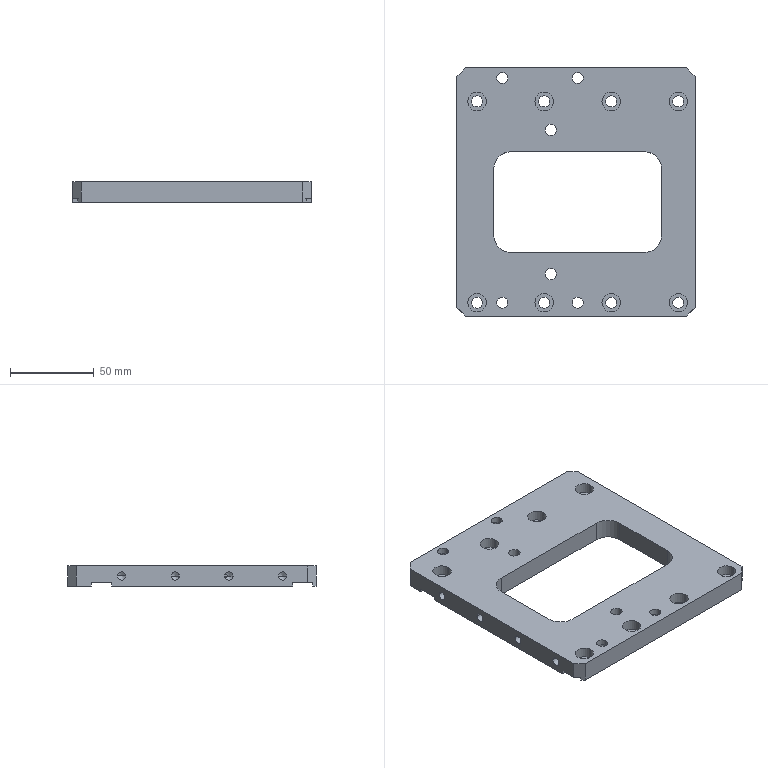Component | SolidWorks | 17081801-804-013A-1 | 1 solid | 106 faces | box 142 x 148 x 12 mm | volume 162736 mm3 | cylinder 64 | plane 34 | cone 8 | commonest cylinder face diameters 11 x24 6.6 x24 5 x8 6.8 x4 20 x4 | material AL6061
build123d program:
from build123d import *

# Parameters (mm, degrees)
SKETCH1_W                                       = 136
SKETCH1_H                                       = 140
BOSS_EXTRUDE1_DEPTH                             = 6
M6_HEX_SOCKET_HEAD_CAP_SCREW_CBORE1_D           = 6.6
M6_HEX_SOCKET_HEAD_CAP_SCREW_CBORE1_DEPTH       = 13
M6_HEX_SOCKET_HEAD_CAP_SCREW_CBORE1_CBORE_D     = 11
M6_HEX_SOCKET_HEAD_CAP_SCREW_CBORE1_CBORE_DEPTH = 6.4
M6_HEX_SOCKET_HEAD_CAP_SCREW_CBORE1_TIP         = 1.983
SKETCH12_W                                      = 136
SKETCH12_H                                      = 12
BOSS_EXTRUDE2_DEPTH                             = 2
M6_TAPPED_HOLE1_D                               = 5
M6_TAPPED_HOLE1_DEPTH                           = 13
M6_TAPPED_HOLE1_TIP                             = 1.502
SKETCH9_W                                       = 12
SKETCH9_H                                       = 180
CUT_EXTRUDE2_DEPTH                              = 2
SKETCH13_W                                      = 142
SKETCH13_H                                      = 12
BOSS_EXTRUDE3_DEPTH                             = 12
M6_HEX_SOCKET_HEAD_CAP_SCREW_CBORE2_AT_2_COUNT  = 2
M6_HEX_SOCKET_HEAD_CAP_SCREW_CBORE2_AT_2_PITCH  = 134
LPATTERN1_COUNT                                 = 2
LPATTERN1_PITCH                                 = 45
SKETCH8_W                                       = 60
SKETCH8_H                                       = 100
CUT_EXTRUDE1_DEPTH                              = 109.296
FILLET1_R                                       = 10
CHAMFER3_SIZE                                   = 5
M8_TAPPED_HOLE1_D                               = 6.8


with BuildPart() as part:
    # Sketch1 → Boss-Extrude1 (new, symmetric)
    with BuildSketch(Plane(origin=(0, 0, 0), x_dir=(1, 0, 0), z_dir=(0, 1, 0))):
        Rectangle(SKETCH1_W, SKETCH1_H)
    extrude(amount=BOSS_EXTRUDE1_DEPTH, both=True)

    # M6 Hex Socket Head Cap Screw CBORE1
    with Locations(Plane(origin=(0, 6, 0), x_dir=(1, 0, 0), z_dir=(0, 1, 0))):
        with Locations((-60, -60), (60, -60), (60, -20), (60, 20), (60, 60), (-60, 60), (-60, 20), (-60, -20)):
            CounterBoreHole(M6_HEX_SOCKET_HEAD_CAP_SCREW_CBORE1_D / 2, M6_HEX_SOCKET_HEAD_CAP_SCREW_CBORE1_CBORE_D / 2, M6_HEX_SOCKET_HEAD_CAP_SCREW_CBORE1_CBORE_DEPTH, depth=M6_HEX_SOCKET_HEAD_CAP_SCREW_CBORE1_DEPTH)
            with Locations((0, 0, -(M6_HEX_SOCKET_HEAD_CAP_SCREW_CBORE1_DEPTH + M6_HEX_SOCKET_HEAD_CAP_SCREW_CBORE1_TIP / 2))):  # 118° drill point
                Cone(0, M6_HEX_SOCKET_HEAD_CAP_SCREW_CBORE1_D / 2, M6_HEX_SOCKET_HEAD_CAP_SCREW_CBORE1_TIP, mode=Mode.SUBTRACT)

    # Sketch12 → Boss-Extrude2 (add)
    with BuildSketch(Plane(origin=(0, 0, -70), x_dir=(-1, 0, 0), z_dir=(0, 0, -1))):
        Rectangle(SKETCH12_W, SKETCH12_H)
    extrude(amount=BOSS_EXTRUDE2_DEPTH)

    # M6 Tapped Hole1
    with Locations(Plane(origin=(0, 0, -72), x_dir=(-1, 0, 0), z_dir=(0, 0, -1))):
        with Locations((48, 0), (16, 0), (-16, 0), (-48, 0)):
            Hole(M6_TAPPED_HOLE1_D / 2, depth=M6_TAPPED_HOLE1_DEPTH)
            with Locations((0, 0, -(M6_TAPPED_HOLE1_DEPTH + M6_TAPPED_HOLE1_TIP / 2))):  # 118° drill point
                Cone(0, M6_TAPPED_HOLE1_D / 2, M6_TAPPED_HOLE1_TIP, mode=Mode.SUBTRACT)

    # Sketch9 → Cut-Extrude2 (cut)
    with BuildSketch(Plane.XZ.offset(6)):
        with Locations((60, 0)):
            Rectangle(SKETCH9_W, SKETCH9_H)
        with Locations((-60, 0)):
            Rectangle(SKETCH9_W, SKETCH9_H)
    extrude(amount=-CUT_EXTRUDE2_DEPTH, mode=Mode.SUBTRACT)

    # Sketch13 → Boss-Extrude3 (add)
    with BuildSketch(Plane(origin=(68, 0, 0), x_dir=(0, 0, -1), z_dir=(1, 0, 0))):
        with Locations((1, 0)):
            Rectangle(SKETCH13_W, SKETCH13_H)
    extrude(amount=BOSS_EXTRUDE3_DEPTH)

    # Sketch6 → M6 Hex Socket Head Cap Screw CBORE2 (revolve, cut)
    with BuildSketch(Plane(origin=(-60, -6, -45), x_dir=(0, 0, -1), z_dir=(1, 0, 0))):
        Polygon((0, 0), (0, 14.983), (3.3, 13), (3.3, 8.4), (5.5, 8.4), (5.5, 0), align=None)
    m6_hex_socket_head_cap_screw_cbore2 = revolve(axis=Axis((-60, -12.35, -45), (0, 1, 0)), mode=Mode.SUBTRACT)

    # M6 Hex Socket Head Cap Screw CBORE2 at 2: M6 Hex Socket Head Cap Screw CBORE2 ×2
    with Locations(*[(i * M6_HEX_SOCKET_HEAD_CAP_SCREW_CBORE2_AT_2_PITCH, 0, 0) for i in range(1, M6_HEX_SOCKET_HEAD_CAP_SCREW_CBORE2_AT_2_COUNT)]):
        add(m6_hex_socket_head_cap_screw_cbore2, mode=Mode.SUBTRACT)

    # LPattern1: M6 Hex Socket Head Cap Screw CBORE2 ×2
    with Locations(*[(0, 0, i * LPATTERN1_PITCH) for i in range(1, LPATTERN1_COUNT)]):
        add(m6_hex_socket_head_cap_screw_cbore2, mode=Mode.SUBTRACT)

    # LPattern1 copy 1 sketch → LPattern1 copy 1 (revolve, cut)
    with BuildSketch(Plane(origin=(74, -6, 0), x_dir=(0, 0, -1), z_dir=(1, 0, 0))):
        Polygon((0, 0), (0, 14.983), (3.3, 13), (3.3, 8.4), (5.5, 8.4), (5.5, 0), align=None)
    revolve(axis=Axis((74, -12.35, 0), (0, 1, 0)), mode=Mode.SUBTRACT)

    # Sketch8 → Cut-Extrude1 (cut, through all)
    with BuildSketch(Plane.XZ.offset(6)):
        Rectangle(SKETCH8_W, SKETCH8_H)
    extrude(amount=-CUT_EXTRUDE1_DEPTH, mode=Mode.SUBTRACT)

    # Fillet1
    fillet1_edges = [part.edges().sort_by_distance(p)[0] for p in [
        (-30, 0, -50),
        (-30, 0, 50),
        (30, 0, 50),
        (30, 0, -50),
    ]]
    fillet(fillet1_edges, radius=FILLET1_R)

    # Chamfer3
    chamfer3_edges = [part.edges().sort_by_distance(p)[0] for p in [
        (80, 0, 70),
        (80, 0, -72),
        (-68, 0, 70),
        (-68, 0, -72),
    ]]
    chamfer(chamfer3_edges, length=CHAMFER3_SIZE)

    # M8 Tapped Hole1 (through all)
    with Locations(Plane(origin=(0, 6, 0), x_dir=(1, 0, 0), z_dir=(0, 1, 0))):
        with Locations((-43, 16), (43, 16)):
            Hole(M8_TAPPED_HOLE1_D / 2)


solid = part.part

# Placed as in the assembly
solid = solid.moved(Location((-44.5, 2034.4, 226), (90, 90, 0)))